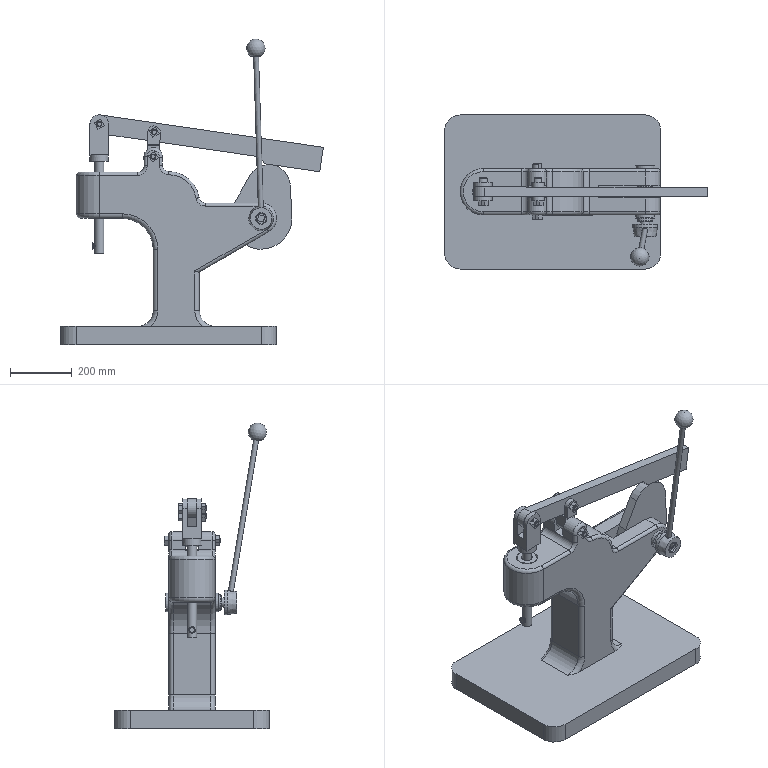Assembly | NX | mm | 20 component files | 20 solids | 532 faces | box 851.72 x 500 x 991.72 mm | volume 46389758 mm3 | plane 157 | cylinder 152 | other 100 | spline 61 | cone 39 | torus 22 | sphere 1 | commonest cylinder face diameters 20 x22 16.625 x20 30 x19 8 x16 60 x8 100 x8 16 x7 14 x7
Bill of materials:
unnamed part 1 | 1 |  | Bracket on a flat rectangular base plate with rounded corners. A single upright web rises from the plate and curves into an overhanging upper arm, which ends in a block with a vertical hole. A small rounded tab with a hole sits on top. A slotted, fork-like arm runs diagonally from the web and has a cross hole near its rounded end.
unnamed part 2 | 2 |  | Flanged cylindrical sleeve (bushing-like) with a plain through bore, a thin flange at one end and a small chamfer on the outer edge at the other end.
unnamed part 3 | 1 |  | Screw-like part with a short cylindrical head carrying about 20 radial teeth or flutes with chamfered edges. Below the head is a plain neck with a fillet, then a threaded-looking shank with a chamfered tip.
unnamed part 4 | 1 |  | Long slender cylindrical rod with a fork (clevis-like) end. The fork has two parallel lugs with rounded tops and a shared cross hole, and a short collar step where it meets the rod.
unnamed part 5 | 2 |  | Shouldered pin or bolt-like part. It has a cylindrical head with two parallel flats and a chamfer, a long smooth cylindrical shoulder, a short reduced neck, and a smaller threaded-looking end.
unnamed part 6 | 1 |  | Very long, thin cylindrical rod with short reduced-diameter ends at both ends that look threaded.
unnamed part 7 | 1 |  | Stepped shaft. It has a long cylindrical main body with an elongated slot (keyway-like pocket), a thin raised flange collar, a short smaller step, and a square drive end.
unnamed part 8 | 1 |  | Short collar or hub with a square through hole and a counterbore at one face. The outer surface combines a cylindrical band and a tapered conical section. A radial hole runs into the side wall.
unnamed part 9 | 1 |  | Long shouldered pin or bolt-like part with a cylindrical head that is chamfered and has flats, a long smooth slender shank, and a short reduced threaded-looking end.
unnamed part 10 | 1 |  | Clevis or fork block. Two parallel lugs with rounded ends, each with a cross hole, are separated by a rectangular slot. They join a solid tongue section with a rounded end and its own parallel hole.
unnamed part 11 | 1 |  | Flat plate of uniform thickness with a teardrop or egg-shaped profile, like a cam. It has a small round bore with a single rectangular keyway notch.
unnamed part 12 | 1 |  | Near-spherical solid ball. Some views show a small flattened region or truncation on one side.
unnamed part 13 | 1 |  | Long, thin, flat bar of constant thickness. One end is rounded and the other is cut square at a slight angle. There are two small round through-holes near the rounded end, and the bar widens in a short angled step near the square end.
unnamed part 14 | 1 |  | Flanged cylindrical sleeve (bushing-like) with a plain through-bore. A thin, wider flange sits at one end, a longer straight cylindrical body follows, and the other end has a small chamfer.
unnamed part 15 | 3 |  | Square block with a central threaded through-hole, resembling a square nut. It is noticeably thicker than a typical thin nut, and its edges look sharp with no chamfers.
unnamed part 16 | 1 |  | Solid stadium-shaped (obround) prism with two rounded ends, flat top and bottom faces, and small chamfers around the edges of both flat faces. It resembles a round-ended parallel key.
Mates:
1. fix | machine_base 1 component
2. concentric | control_rod 1 edge | handle_knob 1 edge
3. concentric | twist_wheel 1 edge | control_rod 1 edge
4. touch align | spindle 1 face | machine_base 1 face
5. touch align | twist_wheel 1 face | spindle 1 face
6. touch align | twist_wheel 1 face | spindle 1 face
7. touch align | twist_wheel 1 face | spindle 1 face
8. concentric | long_pin 1 edge | machine_base 1 edge
9. touch align | shaft_key 1 face | spindle 1 face
10. touch align | shaft_key 1 face | spindle 1 face
11. touch align | shaft_key 1 face | spindle 1 face
12. touch align | cam 1 face | spindle 1 face
13. touch align | cam 1 face | shaft_key 1 face
14. distance | machine_base 1 face | cam 1 face
15. touch align | machine_base 1 face | spindle_sleeve 2 face
16. touch align | spindle_sleeve 2 face | machine_base 1 face
17. touch align | spindle_sleeve 1 face | machine_base 1 face
18. touch align | spindle_sleeve 1 face | machine_base 1 face
19. touch align | spindle 1 face | spindle_sleeve 1 face
20. touch align | pressure_shaft 1 face | machine_base 1 face
21. touch align | swing_bracket 1 face | long_pin 1 face
22. touch align | power_rod 1 face | pressure_shaft 1 face
23. concentric | short_pin 2 edge | swing_bracket 1 edge
24. concentric | square_nut 3 edge | long_pin 1 edge
25. concentric | square_nut 2 edge | short_pin 2 edge
26. touch align | swing_bracket 1 face | machine_base 1 face
27. touch align | short_pin 2 face | power_rod 1 face
28. touch align | power_rod 1 face | cam 1 face
29. touch align | pressure_bushing 1 face | pressure_shaft 1 face
30. touch align | machine_base 1 face | pressure_bushing 1 face
31. touch align | pressure_shaft 1 face | power_rod 1 face
32. concentric | short_pin 1 edge | pressure_shaft 1 edge
33. concentric | square_nut 1 edge | short_pin 1 edge
34. touch align | locking_screw 1 face | pressure_shaft 1 face
35. touch align | locking_screw 1 face | pressure_shaft 1 face